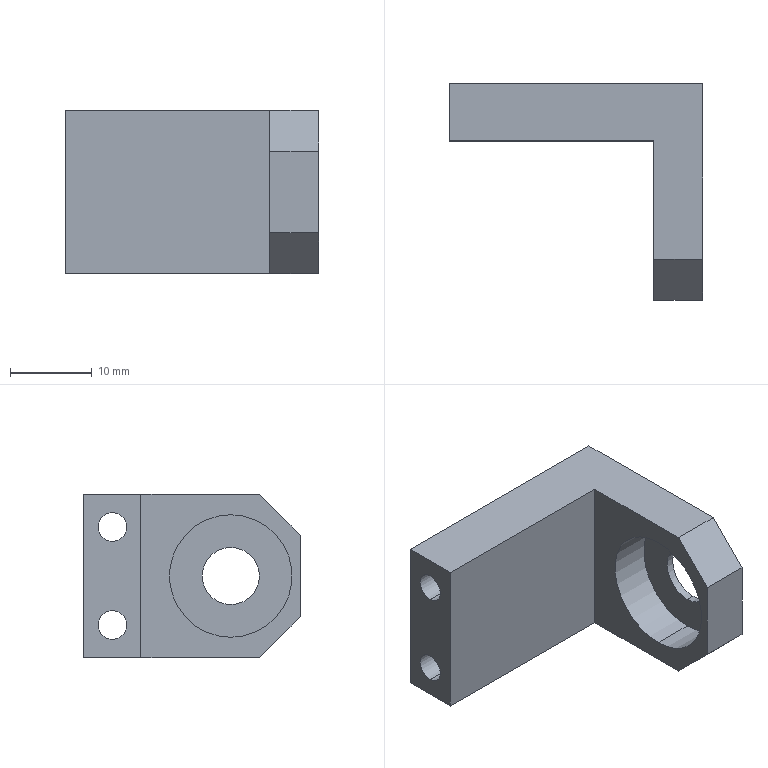Component | SolidWorks | AS-011-JG0130-1 | 1 solid | 19 faces | box 31 x 26.5 x 20 mm | volume 5011 mm3 | plane 11 | cylinder 8 | commonest cylinder face diameters 3.5 x4 15 x2 7 x2
build123d program:
from build123d import *

# Parameters (mm, degrees)
BOSS_EXTRUDE1_DEPTH = 20
SKETCH2_R           = 3.5
SKETCH2_R_2         = 1.75
CUT_EXTRUDE1_DEPTH  = 42
SKETCH5_R           = 7.5
CUT_EXTRUDE2_DEPTH  = 5
CHAMFER1_SIZE       = 5


with BuildPart() as part:
    # Sketch1 → Boss-Extrude1 (new body)
    with BuildSketch(Plane.XY):
        Polygon((-6, -7), (-6, -26.5), (0, -26.5), (0, 0), (-31, 0), (-31, -7), align=None)
    extrude(amount=-BOSS_EXTRUDE1_DEPTH)

    # Sketch2 → Cut-Extrude1 (cut)
    with BuildSketch(Plane(origin=(0, 0, 0), x_dir=(0, 0, -1), z_dir=(1, 0, 0))):
        with Locations((10, -18)):
            Circle(SKETCH2_R)
        with Locations((4, -3.5)):
            Circle(SKETCH2_R_2)
        with Locations((16, -3.5)):
            Circle(SKETCH2_R_2)
    extrude(amount=-CUT_EXTRUDE1_DEPTH, mode=Mode.SUBTRACT)

    # Sketch5 → Cut-Extrude2 (cut)
    with BuildSketch(Plane.ZY.offset(6)):
        with Locations((-10, -18)):
            Circle(SKETCH5_R)
    extrude(amount=-CUT_EXTRUDE2_DEPTH, mode=Mode.SUBTRACT)

    # Chamfer1
    chamfer1_edges = [part.edges().sort_by_distance(p)[0] for p in [
        (-3, -26.5, -20),
        (-3, -26.5, 0),
    ]]
    chamfer(chamfer1_edges, length=CHAMFER1_SIZE)


solid = part.part
STEP:
#1=COLOUR_RGB('',0.7922,0.8196,0.9333);
#2=FILL_AREA_STYLE_COLOUR('',#1);
#3=FILL_AREA_STYLE('',(#2));
#4=SURFACE_STYLE_FILL_AREA(#3);
#5=SURFACE_SIDE_STYLE('',(#4));
#6=SURFACE_STYLE_USAGE(.BOTH.,#5);
#7=PRESENTATION_STYLE_ASSIGNMENT((#6));
#8=CARTESIAN_POINT('',(-0.03937,-0.7087,-0.689));
#9=VERTEX_POINT('',#8);
#10=CARTESIAN_POINT('',(-0.03937,-0.7087,-0.09843));
#11=VERTEX_POINT('',#10);
#12=CARTESIAN_POINT('',(-0.03937,-0.7087,-0.3937));
#13=DIRECTION('',(-1.,0.,0.));
#14=DIRECTION('',(0.,0.,1.));
#15=AXIS2_PLACEMENT_3D('',#12,#13,#14);
#16=CIRCLE('',#15,0.2953);
#17=EDGE_CURVE('',#9,#11,#16,.T.);
#18=ORIENTED_EDGE('',*,*,#17,.F.);
#19=CARTESIAN_POINT('',(-0.2362,-0.7087,-0.689));
#20=VERTEX_POINT('',#19);
#21=CARTESIAN_POINT('',(-0.03937,-0.7087,-0.689));
#22=DIRECTION('',(-1.,0.,0.));
#23=VECTOR('',#22,39.37);
#24=LINE('',#21,#23);
#25=EDGE_CURVE('',#9,#20,#24,.T.);
#26=ORIENTED_EDGE('',*,*,#25,.T.);
#27=CARTESIAN_POINT('',(-0.2362,-0.7087,-0.09843));
#28=VERTEX_POINT('',#27);
#29=CARTESIAN_POINT('',(-0.2362,-0.7087,-0.3937));
#30=DIRECTION('',(-1.,0.,0.));
#31=DIRECTION('',(0.,0.,1.));
#32=AXIS2_PLACEMENT_3D('',#29,#30,#31);
#33=CIRCLE('',#32,0.2953);
#34=EDGE_CURVE('',#20,#28,#33,.T.);
#35=ORIENTED_EDGE('',*,*,#34,.T.);
#36=CARTESIAN_POINT('',(-0.03937,-0.7087,-0.09843));
#37=DIRECTION('',(-1.,0.,0.));
#38=VECTOR('',#37,39.37);
#39=LINE('',#36,#38);
#40=EDGE_CURVE('',#11,#28,#39,.T.);
#41=ORIENTED_EDGE('',*,*,#40,.F.);
#42=EDGE_LOOP('',(#18,#26,#35,#41));
#43=FACE_OUTER_BOUND('',#42,.T.);
#44=CARTESIAN_POINT('',(-0.03937,-0.7087,-0.3937));
#45=DIRECTION('',(-1.,0.,0.));
#46=DIRECTION('',(0.,0.,1.));
#47=AXIS2_PLACEMENT_3D('',#44,#45,#46);
#48=CYLINDRICAL_SURFACE('',#47,0.2953);
#49=ADVANCED_FACE('',(#43),#48,.F.);
#50=CARTESIAN_POINT('',(-1.22,-0.1378,-0.6988));
#51=VERTEX_POINT('',#50);
#52=CARTESIAN_POINT('',(-1.22,-0.1378,-0.561));
#53=VERTEX_POINT('',#52);
#54=CARTESIAN_POINT('',(-1.22,-0.1378,-0.6299));
#55=DIRECTION('',(-1.,0.,0.));
#56=DIRECTION('',(0.,0.,1.));
#57=AXIS2_PLACEMENT_3D('',#54,#55,#56);
#58=CIRCLE('',#57,0.0689);
#59=EDGE_CURVE('',#51,#53,#58,.T.);
#60=ORIENTED_EDGE('',*,*,#59,.T.);
#61=CARTESIAN_POINT('',(0.,-0.1378,-0.561));
#62=VERTEX_POINT('',#61);
#63=CARTESIAN_POINT('',(-1.654,-0.1378,-0.561));
#64=DIRECTION('',(1.,0.,0.));
#65=VECTOR('',#64,39.37);
#66=LINE('',#63,#65);
#67=EDGE_CURVE('',#53,#62,#66,.T.);
#68=ORIENTED_EDGE('',*,*,#67,.T.);
#69=CARTESIAN_POINT('',(0.,-0.1378,-0.6988));
#70=VERTEX_POINT('',#69);
#71=CARTESIAN_POINT('',(0.,-0.1378,-0.6299));
#72=DIRECTION('',(1.,0.,0.));
#73=DIRECTION('',(0.,0.,-1.));
#74=AXIS2_PLACEMENT_3D('',#71,#72,#73);
#75=CIRCLE('',#74,0.0689);
#76=EDGE_CURVE('',#62,#70,#75,.T.);
#77=ORIENTED_EDGE('',*,*,#76,.T.);
#78=CARTESIAN_POINT('',(-1.654,-0.1378,-0.6988));
#79=DIRECTION('',(1.,0.,0.));
#80=VECTOR('',#79,39.37);
#81=LINE('',#78,#80);
#82=EDGE_CURVE('',#51,#70,#81,.T.);
#83=ORIENTED_EDGE('',*,*,#82,.F.);
#84=EDGE_LOOP('',(#60,#68,#77,#83));
#85=FACE_OUTER_BOUND('',#84,.T.);
#86=CARTESIAN_POINT('',(-1.654,-0.1378,-0.6299));
#87=DIRECTION('',(1.,0.,0.));
#88=DIRECTION('',(0.,0.,-1.));
#89=AXIS2_PLACEMENT_3D('',#86,#87,#88);
#90=CYLINDRICAL_SURFACE('',#89,0.0689);
#91=ADVANCED_FACE('',(#85),#90,.F.);
#92=CARTESIAN_POINT('',(-1.22,-0.1378,-0.2264));
#93=VERTEX_POINT('',#92);
#94=CARTESIAN_POINT('',(-1.22,-0.1378,-0.08858));
#95=VERTEX_POINT('',#94);
#96=CARTESIAN_POINT('',(-1.22,-0.1378,-0.1575));
#97=DIRECTION('',(-1.,0.,0.));
#98=DIRECTION('',(0.,0.,1.));
#99=AXIS2_PLACEMENT_3D('',#96,#97,#98);
#100=CIRCLE('',#99,0.0689);
#101=EDGE_CURVE('',#93,#95,#100,.T.);
#102=ORIENTED_EDGE('',*,*,#101,.T.);
#103=CARTESIAN_POINT('',(0.,-0.1378,-0.08858));
#104=VERTEX_POINT('',#103);
#105=CARTESIAN_POINT('',(-1.654,-0.1378,-0.08858));
#106=DIRECTION('',(1.,0.,0.));
#107=VECTOR('',#106,39.37);
#108=LINE('',#105,#107);
#109=EDGE_CURVE('',#95,#104,#108,.T.);
#110=ORIENTED_EDGE('',*,*,#109,.T.);
#111=CARTESIAN_POINT('',(0.,-0.1378,-0.2264));
#112=VERTEX_POINT('',#111);
#113=CARTESIAN_POINT('',(0.,-0.1378,-0.1575));
#114=DIRECTION('',(1.,0.,0.));
#115=DIRECTION('',(0.,0.,-1.));
#116=AXIS2_PLACEMENT_3D('',#113,#114,#115);
#117=CIRCLE('',#116,0.0689);
#118=EDGE_CURVE('',#104,#112,#117,.T.);
#119=ORIENTED_EDGE('',*,*,#118,.T.);
#120=CARTESIAN_POINT('',(-1.654,-0.1378,-0.2264));
#121=DIRECTION('',(1.,0.,0.));
#122=VECTOR('',#121,39.37);
#123=LINE('',#120,#122);
#124=EDGE_CURVE('',#93,#112,#123,.T.);
#125=ORIENTED_EDGE('',*,*,#124,.F.);
#126=EDGE_LOOP('',(#102,#110,#119,#125));
#127=FACE_OUTER_BOUND('',#126,.T.);
#128=CARTESIAN_POINT('',(-1.654,-0.1378,-0.1575));
#129=DIRECTION('',(1.,0.,0.));
#130=DIRECTION('',(0.,0.,-1.));
#131=AXIS2_PLACEMENT_3D('',#128,#129,#130);
#132=CYLINDRICAL_SURFACE('',#131,0.0689);
#133=ADVANCED_FACE('',(#127),#132,.F.);
#134=CARTESIAN_POINT('',(-0.03937,-0.7087,-0.2559));
#135=VERTEX_POINT('',#134);
#136=CARTESIAN_POINT('',(-0.03937,-0.7087,-0.5315));
#137=VERTEX_POINT('',#136);
#138=CARTESIAN_POINT('',(-0.03937,-0.7087,-0.3937));
#139=DIRECTION('',(1.,0.,0.));
#140=DIRECTION('',(0.,0.,1.));
#141=AXIS2_PLACEMENT_3D('',#138,#139,#140);
#142=CIRCLE('',#141,0.1378);
#143=EDGE_CURVE('',#135,#137,#142,.T.);
#144=ORIENTED_EDGE('',*,*,#143,.F.);
#145=CARTESIAN_POINT('',(0.,-0.7087,-0.2559));
#146=VERTEX_POINT('',#145);
#147=CARTESIAN_POINT('',(-1.654,-0.7087,-0.2559));
#148=DIRECTION('',(1.,0.,0.));
#149=VECTOR('',#148,39.37);
#150=LINE('',#147,#149);
#151=EDGE_CURVE('',#135,#146,#150,.T.);
#152=ORIENTED_EDGE('',*,*,#151,.T.);
#153=CARTESIAN_POINT('',(0.,-0.7087,-0.5315));
#154=VERTEX_POINT('',#153);
#155=CARTESIAN_POINT('',(0.,-0.7087,-0.3937));
#156=DIRECTION('',(1.,0.,0.));
#157=DIRECTION('',(0.,0.,-1.));
#158=AXIS2_PLACEMENT_3D('',#155,#156,#157);
#159=CIRCLE('',#158,0.1378);
#160=EDGE_CURVE('',#146,#154,#159,.T.);
#161=ORIENTED_EDGE('',*,*,#160,.T.);
#162=CARTESIAN_POINT('',(-1.654,-0.7087,-0.5315));
#163=DIRECTION('',(1.,0.,0.));
#164=VECTOR('',#163,39.37);
#165=LINE('',#162,#164);
#166=EDGE_CURVE('',#137,#154,#165,.T.);
#167=ORIENTED_EDGE('',*,*,#166,.F.);
#168=EDGE_LOOP('',(#144,#152,#161,#167));
#169=FACE_OUTER_BOUND('',#168,.T.);
#170=CARTESIAN_POINT('',(-1.654,-0.7087,-0.3937));
#171=DIRECTION('',(1.,0.,0.));
#172=DIRECTION('',(0.,0.,-1.));
#173=AXIS2_PLACEMENT_3D('',#170,#171,#172);
#174=CYLINDRICAL_SURFACE('',#173,0.1378);
#175=ADVANCED_FACE('',(#169),#174,.F.);
#176=ORIENTED_EDGE('',*,*,#151,.F.);
#177=CARTESIAN_POINT('',(-0.03937,-0.7087,-0.3937));
#178=DIRECTION('',(1.,0.,0.));
#179=DIRECTION('',(0.,0.,1.));
#180=AXIS2_PLACEMENT_3D('',#177,#178,#179);
#181=CIRCLE('',#180,0.1378);
#182=EDGE_CURVE('',#137,#135,#181,.T.);
#183=ORIENTED_EDGE('',*,*,#182,.F.);
#184=ORIENTED_EDGE('',*,*,#166,.T.);
#185=CARTESIAN_POINT('',(0.,-0.7087,-0.3937));
#186=DIRECTION('',(1.,0.,0.));
#187=DIRECTION('',(0.,0.,-1.));
#188=AXIS2_PLACEMENT_3D('',#185,#186,#187);
#189=CIRCLE('',#188,0.1378);
#190=EDGE_CURVE('',#154,#146,#189,.T.);
#191=ORIENTED_EDGE('',*,*,#190,.T.);
#192=EDGE_LOOP('',(#176,#183,#184,#191));
#193=FACE_OUTER_BOUND('',#192,.T.);
#194=CARTESIAN_POINT('',(-1.654,-0.7087,-0.3937));
#195=DIRECTION('',(1.,0.,0.));
#196=DIRECTION('',(0.,0.,-1.));
#197=AXIS2_PLACEMENT_3D('',#194,#195,#196);
#198=CYLINDRICAL_SURFACE('',#197,0.1378);
#199=ADVANCED_FACE('',(#193),#198,.F.);
#200=CARTESIAN_POINT('',(-1.22,-0.2756,0.));
#201=VERTEX_POINT('',#200);
#202=CARTESIAN_POINT('',(-0.2362,-0.2756,0.));
#203=VERTEX_POINT('',#202);
#204=CARTESIAN_POINT('',(-1.22,-0.2756,0.));
#205=DIRECTION('',(1.,0.,0.));
#206=VECTOR('',#205,39.37);
#207=LINE('',#204,#206);
#208=EDGE_CURVE('',#201,#203,#207,.T.);
#209=ORIENTED_EDGE('',*,*,#208,.F.);
#210=CARTESIAN_POINT('',(-1.22,-0.2756,-0.7874));
#211=VERTEX_POINT('',#210);
#212=CARTESIAN_POINT('',(-1.22,-0.2756,-0.7874));
#213=DIRECTION('',(0.,0.,1.));
#214=VECTOR('',#213,39.37);
#215=LINE('',#212,#214);
#216=EDGE_CURVE('',#211,#201,#215,.T.);
#217=ORIENTED_EDGE('',*,*,#216,.F.);
#218=CARTESIAN_POINT('',(-0.2362,-0.2756,-0.7874));
#219=VERTEX_POINT('',#218);
#220=CARTESIAN_POINT('',(-1.22,-0.2756,-0.7874));
#221=DIRECTION('',(1.,0.,0.));
#222=VECTOR('',#221,39.37);
#223=LINE('',#220,#222);
#224=EDGE_CURVE('',#211,#219,#223,.T.);
#225=ORIENTED_EDGE('',*,*,#224,.T.);
#226=CARTESIAN_POINT('',(-0.2362,-0.2756,-0.7874));
#227=DIRECTION('',(0.,0.,1.));
#228=VECTOR('',#227,39.37);
#229=LINE('',#226,#228);
#230=EDGE_CURVE('',#219,#203,#229,.T.);
#231=ORIENTED_EDGE('',*,*,#230,.T.);
#232=EDGE_LOOP('',(#209,#217,#225,#231));
#233=FACE_OUTER_BOUND('',#232,.T.);
#234=CARTESIAN_POINT('',(-1.22,-0.2756,-0.7874));
#235=DIRECTION('',(0.,-1.,0.));
#236=DIRECTION('',(0.,0.,-1.));
#237=AXIS2_PLACEMENT_3D('',#234,#235,#236);
#238=PLANE('',#237);
#239=ADVANCED_FACE('',(#233),#238,.T.);
#240=ORIENTED_EDGE('',*,*,#59,.F.);
#241=CARTESIAN_POINT('',(-1.22,-0.1378,-0.6299));
#242=DIRECTION('',(-1.,0.,0.));
#243=DIRECTION('',(0.,0.,1.));
#244=AXIS2_PLACEMENT_3D('',#241,#242,#243);
#245=CIRCLE('',#244,0.0689);
#246=EDGE_CURVE('',#53,#51,#245,.T.);
#247=ORIENTED_EDGE('',*,*,#246,.F.);
#248=EDGE_LOOP('',(#240,#247));
#249=FACE_BOUND('',#248,.T.);
#250=ORIENTED_EDGE('',*,*,#101,.F.);
#251=CARTESIAN_POINT('',(-1.22,-0.1378,-0.1575));
#252=DIRECTION('',(-1.,0.,0.));
#253=DIRECTION('',(0.,0.,1.));
#254=AXIS2_PLACEMENT_3D('',#251,#252,#253);
#255=CIRCLE('',#254,0.0689);
#256=EDGE_CURVE('',#95,#93,#255,.T.);
#257=ORIENTED_EDGE('',*,*,#256,.F.);
#258=EDGE_LOOP('',(#250,#257));
#259=FACE_BOUND('',#258,.T.);
#260=CARTESIAN_POINT('',(-1.22,0.,0.));
#261=VERTEX_POINT('',#260);
#262=CARTESIAN_POINT('',(-1.22,-0.2756,0.));
#263=DIRECTION('',(0.,-1.,0.));
#264=VECTOR('',#263,39.37);
#265=LINE('',#262,#264);
#266=EDGE_CURVE('',#261,#201,#265,.T.);
#267=ORIENTED_EDGE('',*,*,#266,.F.);
#268=CARTESIAN_POINT('',(-1.22,0.,-0.7874));
#269=VERTEX_POINT('',#268);
#270=CARTESIAN_POINT('',(-1.22,0.,-0.7874));
#271=DIRECTION('',(0.,0.,1.));
#272=VECTOR('',#271,39.37);
#273=LINE('',#270,#272);
#274=EDGE_CURVE('',#269,#261,#273,.T.);
#275=ORIENTED_EDGE('',*,*,#274,.F.);
#276=CARTESIAN_POINT('',(-1.22,-0.2756,-0.7874));
#277=DIRECTION('',(0.,-1.,0.));
#278=VECTOR('',#277,39.37);
#279=LINE('',#276,#278);
#280=EDGE_CURVE('',#269,#211,#279,.T.);
#281=ORIENTED_EDGE('',*,*,#280,.T.);
#282=ORIENTED_EDGE('',*,*,#216,.T.);
#283=EDGE_LOOP('',(#267,#275,#281,#282));
#284=FACE_OUTER_BOUND('',#283,.T.);
#285=CARTESIAN_POINT('',(-1.22,-0.2756,-0.7874));
#286=DIRECTION('',(-1.,0.,0.));
#287=DIRECTION('',(0.,0.,1.));
#288=AXIS2_PLACEMENT_3D('',#285,#286,#287);
#289=PLANE('',#288);
#290=ADVANCED_FACE('',(#249,#259,#284),#289,.T.);
#291=CARTESIAN_POINT('',(0.,0.,0.));
#292=VERTEX_POINT('',#291);
#293=CARTESIAN_POINT('',(0.,0.,0.));
#294=DIRECTION('',(-1.,0.,0.));
#295=VECTOR('',#294,39.37);
#296=LINE('',#293,#295);
#297=EDGE_CURVE('',#292,#261,#296,.T.);
#298=ORIENTED_EDGE('',*,*,#297,.F.);
#299=CARTESIAN_POINT('',(0.,0.,-0.7874));
#300=VERTEX_POINT('',#299);
#301=CARTESIAN_POINT('',(0.,0.,-0.7874));
#302=DIRECTION('',(0.,0.,1.));
#303=VECTOR('',#302,39.37);
#304=LINE('',#301,#303);
#305=EDGE_CURVE('',#300,#292,#304,.T.);
#306=ORIENTED_EDGE('',*,*,#305,.F.);
#307=CARTESIAN_POINT('',(0.,0.,-0.7874));
#308=DIRECTION('',(-1.,0.,0.));
#309=VECTOR('',#308,39.37);
#310=LINE('',#307,#309);
#311=EDGE_CURVE('',#300,#269,#310,.T.);
#312=ORIENTED_EDGE('',*,*,#311,.T.);
#313=ORIENTED_EDGE('',*,*,#274,.T.);
#314=EDGE_LOOP('',(#298,#306,#312,#313));
#315=FACE_OUTER_BOUND('',#314,.T.);
#316=CARTESIAN_POINT('',(0.,0.,-0.7874));
#317=DIRECTION('',(0.,1.,0.));
#318=DIRECTION('',(0.,0.,1.));
#319=AXIS2_PLACEMENT_3D('',#316,#317,#318);
#320=PLANE('',#319);
#321=ADVANCED_FACE('',(#315),#320,.T.);
#322=CARTESIAN_POINT('',(0.,-0.1378,-0.6299));
#323=DIRECTION('',(1.,0.,0.));
#324=DIRECTION('',(0.,0.,-1.));
#325=AXIS2_PLACEMENT_3D('',#322,#323,#324);
#326=CIRCLE('',#325,0.0689);
#327=EDGE_CURVE('',#70,#62,#326,.T.);
#328=ORIENTED_EDGE('',*,*,#327,.F.);
#329=ORIENTED_EDGE('',*,*,#76,.F.);
#330=EDGE_LOOP('',(#328,#329));
#331=FACE_BOUND('',#330,.T.);
#332=CARTESIAN_POINT('',(0.,-0.1378,-0.1575));
#333=DIRECTION('',(1.,0.,0.));
#334=DIRECTION('',(0.,0.,-1.));
#335=AXIS2_PLACEMENT_3D('',#332,#333,#334);
#336=CIRCLE('',#335,0.0689);
#337=EDGE_CURVE('',#112,#104,#336,.T.);
#338=ORIENTED_EDGE('',*,*,#337,.F.);
#339=ORIENTED_EDGE('',*,*,#118,.F.);
#340=EDGE_LOOP('',(#338,#339));
#341=FACE_BOUND('',#340,.T.);
#342=ORIENTED_EDGE('',*,*,#190,.F.);
#343=ORIENTED_EDGE('',*,*,#160,.F.);
#344=EDGE_LOOP('',(#342,#343));
#345=FACE_BOUND('',#344,.T.);
#346=CARTESIAN_POINT('',(0.,-1.043,-0.5906));
#347=VERTEX_POINT('',#346);
#348=CARTESIAN_POINT('',(0.,-1.043,-0.1969));
#349=VERTEX_POINT('',#348);
#350=CARTESIAN_POINT('',(0.,-1.043,-0.7874));
#351=DIRECTION('',(0.,0.,1.));
#352=VECTOR('',#351,39.37);
#353=LINE('',#350,#352);
#354=EDGE_CURVE('',#347,#349,#353,.T.);
#355=ORIENTED_EDGE('',*,*,#354,.F.);
#356=CARTESIAN_POINT('',(0.,-0.8465,-0.7874));
#357=VERTEX_POINT('',#356);
#358=CARTESIAN_POINT('',(0.,-0.4232,-1.211));
#359=DIRECTION('',(0.,0.7071,-0.7071));
#360=VECTOR('',#359,39.37);
#361=LINE('',#358,#360);
#362=EDGE_CURVE('',#347,#357,#361,.T.);
#363=ORIENTED_EDGE('',*,*,#362,.T.);
#364=CARTESIAN_POINT('',(0.,0.,-0.7874));
#365=DIRECTION('',(0.,1.,0.));
#366=VECTOR('',#365,39.37);
#367=LINE('',#364,#366);
#368=EDGE_CURVE('',#357,#300,#367,.T.);
#369=ORIENTED_EDGE('',*,*,#368,.T.);
#370=ORIENTED_EDGE('',*,*,#305,.T.);
#371=CARTESIAN_POINT('',(0.,-0.8465,-0.));
#372=VERTEX_POINT('',#371);
#373=CARTESIAN_POINT('',(0.,0.,0.));
#374=DIRECTION('',(0.,1.,0.));
#375=VECTOR('',#374,39.37);
#376=LINE('',#373,#375);
#377=EDGE_CURVE('',#372,#292,#376,.T.);
#378=ORIENTED_EDGE('',*,*,#377,.F.);
#379=CARTESIAN_POINT('',(0.,-0.8169,0.02953));
#380=DIRECTION('',(0.,-0.7071,-0.7071));
#381=VECTOR('',#380,39.37);
#382=LINE('',#379,#381);
#383=EDGE_CURVE('',#372,#349,#382,.T.);
#384=ORIENTED_EDGE('',*,*,#383,.T.);
#385=EDGE_LOOP('',(#355,#363,#369,#370,#378,#384));
#386=FACE_OUTER_BOUND('',#385,.T.);
#387=CARTESIAN_POINT('',(0.,0.,-0.7874));
#388=DIRECTION('',(1.,0.,0.));
#389=DIRECTION('',(0.,0.,-1.));
#390=AXIS2_PLACEMENT_3D('',#387,#388,#389);
#391=PLANE('',#390);
#392=ADVANCED_FACE('',(#331,#341,#345,#386),#391,.T.);
#393=CARTESIAN_POINT('',(-0.2362,-1.043,-0.5906));
#394=VERTEX_POINT('',#393);
#395=CARTESIAN_POINT('',(-0.2362,-1.043,-0.1969));
#396=VERTEX_POINT('',#395);
#397=CARTESIAN_POINT('',(-0.2362,-1.043,-0.7874));
#398=DIRECTION('',(0.,0.,1.));
#399=VECTOR('',#398,39.37);
#400=LINE('',#397,#399);
#401=EDGE_CURVE('',#394,#396,#400,.T.);
#402=ORIENTED_EDGE('',*,*,#401,.F.);
#403=CARTESIAN_POINT('',(0.,-1.043,-0.5906));
#404=DIRECTION('',(1.,0.,0.));
#405=VECTOR('',#404,39.37);
#406=LINE('',#403,#405);
#407=EDGE_CURVE('',#394,#347,#406,.T.);
#408=ORIENTED_EDGE('',*,*,#407,.T.);
#409=ORIENTED_EDGE('',*,*,#354,.T.);
#410=CARTESIAN_POINT('',(-0.2362,-1.043,-0.1969));
#411=DIRECTION('',(-1.,0.,0.));
#412=VECTOR('',#411,39.37);
#413=LINE('',#410,#412);
#414=EDGE_CURVE('',#349,#396,#413,.T.);
#415=ORIENTED_EDGE('',*,*,#414,.T.);
#416=EDGE_LOOP('',(#402,#408,#409,#415));
#417=FACE_OUTER_BOUND('',#416,.T.);
#418=CARTESIAN_POINT('',(0.,-1.043,-0.7874));
#419=DIRECTION('',(0.,-1.,0.));
#420=DIRECTION('',(0.,0.,-1.));
#421=AXIS2_PLACEMENT_3D('',#418,#419,#420);
#422=PLANE('',#421);
#423=ADVANCED_FACE('',(#417),#422,.T.);
#424=CARTESIAN_POINT('',(-0.2362,-0.7087,-0.3937));
#425=DIRECTION('',(-1.,0.,0.));
#426=DIRECTION('',(0.,0.,1.));
#427=AXIS2_PLACEMENT_3D('',#424,#425,#426);
#428=CIRCLE('',#427,0.2953);
#429=EDGE_CURVE('',#28,#20,#428,.T.);
#430=ORIENTED_EDGE('',*,*,#429,.F.);
#431=ORIENTED_EDGE('',*,*,#34,.F.);
#432=EDGE_LOOP('',(#430,#431));
#433=FACE_BOUND('',#432,.T.);
#434=CARTESIAN_POINT('',(-0.2362,-0.8465,-0.7874));
#435=VERTEX_POINT('',#434);
#436=CARTESIAN_POINT('',(-0.2362,-0.2756,-0.7874));
#437=DIRECTION('',(0.,-1.,0.));
#438=VECTOR('',#437,39.37);
#439=LINE('',#436,#438);
#440=EDGE_CURVE('',#219,#435,#439,.T.);
#441=ORIENTED_EDGE('',*,*,#440,.T.);
#442=CARTESIAN_POINT('',(-0.2362,-0.561,-1.073));
#443=DIRECTION('',(0.,-0.7071,0.7071));
#444=VECTOR('',#443,39.37);
#445=LINE('',#442,#444);
#446=EDGE_CURVE('',#435,#394,#445,.T.);
#447=ORIENTED_EDGE('',*,*,#446,.T.);
#448=ORIENTED_EDGE('',*,*,#401,.T.);
#449=CARTESIAN_POINT('',(-0.2362,-0.8465,-0.));
#450=VERTEX_POINT('',#449);
#451=CARTESIAN_POINT('',(-0.2362,-0.9547,-0.1083));
#452=DIRECTION('',(0.,0.7071,0.7071));
#453=VECTOR('',#452,39.37);
#454=LINE('',#451,#453);
#455=EDGE_CURVE('',#396,#450,#454,.T.);
#456=ORIENTED_EDGE('',*,*,#455,.T.);
#457=CARTESIAN_POINT('',(-0.2362,-0.2756,0.));
#458=DIRECTION('',(0.,-1.,0.));
#459=VECTOR('',#458,39.37);
#460=LINE('',#457,#459);
#461=EDGE_CURVE('',#203,#450,#460,.T.);
#462=ORIENTED_EDGE('',*,*,#461,.F.);
#463=ORIENTED_EDGE('',*,*,#230,.F.);
#464=EDGE_LOOP('',(#441,#447,#448,#456,#462,#463));
#465=FACE_OUTER_BOUND('',#464,.T.);
#466=CARTESIAN_POINT('',(-0.2362,-0.2756,-0.7874));
#467=DIRECTION('',(-1.,0.,0.));
#468=DIRECTION('',(0.,0.,1.));
#469=AXIS2_PLACEMENT_3D('',#466,#467,#468);
#470=PLANE('',#469);
#471=ADVANCED_FACE('',(#433,#465),#470,.T.);
#472=ORIENTED_EDGE('',*,*,#368,.F.);
#473=CARTESIAN_POINT('',(0.,-0.8465,-0.7874));
#474=DIRECTION('',(-1.,0.,0.));
#475=VECTOR('',#474,39.37);
#476=LINE('',#473,#475);
#477=EDGE_CURVE('',#357,#435,#476,.T.);
#478=ORIENTED_EDGE('',*,*,#477,.T.);
#479=ORIENTED_EDGE('',*,*,#440,.F.);
#480=ORIENTED_EDGE('',*,*,#224,.F.);
#481=ORIENTED_EDGE('',*,*,#280,.F.);
#482=ORIENTED_EDGE('',*,*,#311,.F.);
#483=EDGE_LOOP('',(#472,#478,#479,#480,#481,#482));
#484=FACE_OUTER_BOUND('',#483,.T.);
#485=CARTESIAN_POINT('',(0.,0.,-0.7874));
#486=DIRECTION('',(0.,0.,-1.));
#487=DIRECTION('',(-1.,0.,0.));
#488=AXIS2_PLACEMENT_3D('',#485,#486,#487);
#489=PLANE('',#488);
#490=ADVANCED_FACE('',(#484),#489,.T.);
#491=ORIENTED_EDGE('',*,*,#461,.T.);
#492=CARTESIAN_POINT('',(0.,-0.8465,0.));
#493=DIRECTION('',(1.,0.,0.));
#494=VECTOR('',#493,39.37);
#495=LINE('',#492,#494);
#496=EDGE_CURVE('',#450,#372,#495,.T.);
#497=ORIENTED_EDGE('',*,*,#496,.T.);
#498=ORIENTED_EDGE('',*,*,#377,.T.);
#499=ORIENTED_EDGE('',*,*,#297,.T.);
#500=ORIENTED_EDGE('',*,*,#266,.T.);
#501=ORIENTED_EDGE('',*,*,#208,.T.);
#502=EDGE_LOOP('',(#491,#497,#498,#499,#500,#501));
#503=FACE_OUTER_BOUND('',#502,.T.);
#504=CARTESIAN_POINT('',(0.,0.,0.));
#505=DIRECTION('',(0.,0.,-1.));
#506=DIRECTION('',(-1.,0.,0.));
#507=AXIS2_PLACEMENT_3D('',#504,#505,#506);
#508=PLANE('',#507);
#509=ADVANCED_FACE('',(#503),#508,.F.);
#510=ORIENTED_EDGE('',*,*,#109,.F.);
#511=ORIENTED_EDGE('',*,*,#256,.T.);
#512=ORIENTED_EDGE('',*,*,#124,.T.);
#513=ORIENTED_EDGE('',*,*,#337,.T.);
#514=EDGE_LOOP('',(#510,#511,#512,#513));
#515=FACE_OUTER_BOUND('',#514,.T.);
#516=CARTESIAN_POINT('',(-1.654,-0.1378,-0.1575));
#517=DIRECTION('',(1.,0.,0.));
#518=DIRECTION('',(0.,0.,-1.));
#519=AXIS2_PLACEMENT_3D('',#516,#517,#518);
#520=CYLINDRICAL_SURFACE('',#519,0.0689);
#521=ADVANCED_FACE('',(#515),#520,.F.);
#522=ORIENTED_EDGE('',*,*,#67,.F.);
#523=ORIENTED_EDGE('',*,*,#246,.T.);
#524=ORIENTED_EDGE('',*,*,#82,.T.);
#525=ORIENTED_EDGE('',*,*,#327,.T.);
#526=EDGE_LOOP('',(#522,#523,#524,#525));
#527=FACE_OUTER_BOUND('',#526,.T.);
#528=CARTESIAN_POINT('',(-1.654,-0.1378,-0.6299));
#529=DIRECTION('',(1.,0.,0.));
#530=DIRECTION('',(0.,0.,-1.));
#531=AXIS2_PLACEMENT_3D('',#528,#529,#530);
#532=CYLINDRICAL_SURFACE('',#531,0.0689);
#533=ADVANCED_FACE('',(#527),#532,.F.);
#534=CARTESIAN_POINT('',(-0.03937,-0.7087,-0.3937));
#535=DIRECTION('',(-1.,0.,0.));
#536=DIRECTION('',(0.,0.,1.));
#537=AXIS2_PLACEMENT_3D('',#534,#535,#536);
#538=CIRCLE('',#537,0.2953);
#539=EDGE_CURVE('',#11,#9,#538,.T.);
#540=ORIENTED_EDGE('',*,*,#539,.T.);
#541=ORIENTED_EDGE('',*,*,#17,.T.);
#542=EDGE_LOOP('',(#540,#541));
#543=FACE_OUTER_BOUND('',#542,.T.);
#544=ORIENTED_EDGE('',*,*,#182,.T.);
#545=ORIENTED_EDGE('',*,*,#143,.T.);
#546=EDGE_LOOP('',(#544,#545));
#547=FACE_BOUND('',#546,.T.);
#548=CARTESIAN_POINT('',(-0.03937,-0.7087,-0.3937));
#549=DIRECTION('',(-1.,0.,0.));
#550=DIRECTION('',(0.,0.,1.));
#551=AXIS2_PLACEMENT_3D('',#548,#549,#550);
#552=PLANE('',#551);
#553=ADVANCED_FACE('',(#543,#547),#552,.T.);
#554=ORIENTED_EDGE('',*,*,#25,.F.);
#555=ORIENTED_EDGE('',*,*,#539,.F.);
#556=ORIENTED_EDGE('',*,*,#40,.T.);
#557=ORIENTED_EDGE('',*,*,#429,.T.);
#558=EDGE_LOOP('',(#554,#555,#556,#557));
#559=FACE_OUTER_BOUND('',#558,.T.);
#560=CARTESIAN_POINT('',(-0.03937,-0.7087,-0.3937));
#561=DIRECTION('',(-1.,0.,0.));
#562=DIRECTION('',(0.,0.,1.));
#563=AXIS2_PLACEMENT_3D('',#560,#561,#562);
#564=CYLINDRICAL_SURFACE('',#563,0.2953);
#565=ADVANCED_FACE('',(#559),#564,.F.);
#566=ORIENTED_EDGE('',*,*,#446,.F.);
#567=ORIENTED_EDGE('',*,*,#477,.F.);
#568=ORIENTED_EDGE('',*,*,#362,.F.);
#569=ORIENTED_EDGE('',*,*,#407,.F.);
#570=EDGE_LOOP('',(#566,#567,#568,#569));
#571=FACE_OUTER_BOUND('',#570,.T.);
#572=CARTESIAN_POINT('',(0.,-1.043,-0.5906));
#573=DIRECTION('',(0.,0.7071,0.7071));
#574=DIRECTION('',(1.,0.,0.));
#575=AXIS2_PLACEMENT_3D('',#572,#573,#574);
#576=PLANE('',#575);
#577=ADVANCED_FACE('',(#571),#576,.F.);
#578=ORIENTED_EDGE('',*,*,#455,.F.);
#579=ORIENTED_EDGE('',*,*,#414,.F.);
#580=ORIENTED_EDGE('',*,*,#383,.F.);
#581=ORIENTED_EDGE('',*,*,#496,.F.);
#582=EDGE_LOOP('',(#578,#579,#580,#581));
#583=FACE_OUTER_BOUND('',#582,.T.);
#584=CARTESIAN_POINT('',(0.,-0.8465,0.));
#585=DIRECTION('',(0.,-0.7071,0.7071));
#586=DIRECTION('',(-1.,0.,0.));
#587=AXIS2_PLACEMENT_3D('',#584,#585,#586);
#588=PLANE('',#587);
#589=ADVANCED_FACE('',(#583),#588,.T.);
#590=CLOSED_SHELL('',(#49,#91,#133,#175,#199,#239,#290,#321,#392,#423,#471,#490,#509,#521,#533,#553,#565,#577,#589));
#591=MANIFOLD_SOLID_BREP('',#590);
#592=STYLED_ITEM('',(#7),#591);
#593=PRESENTATION_LAYER_ASSIGNMENT('','',(#592));
#594=(LENGTH_UNIT()NAMED_UNIT(*)SI_UNIT($,.METRE.));
#595=LENGTH_MEASURE_WITH_UNIT(LENGTH_MEASURE(0.0254),#594);
#596=DIMENSIONAL_EXPONENTS(1.,0.,0.,0.,0.,0.,0.);
#597=(CONVERSION_BASED_UNIT('',#595)LENGTH_UNIT()NAMED_UNIT(#596));
#598=UNCERTAINTY_MEASURE_WITH_UNIT(LENGTH_MEASURE(0.00001),#597,'','');
#599=(NAMED_UNIT(*)PLANE_ANGLE_UNIT()SI_UNIT($,.RADIAN.));
#600=(NAMED_UNIT(*)SI_UNIT($,.STERADIAN.)SOLID_ANGLE_UNIT());
#601=(GEOMETRIC_REPRESENTATION_CONTEXT(3)GLOBAL_UNCERTAINTY_ASSIGNED_CONTEXT((#598))GLOBAL_UNIT_ASSIGNED_CONTEXT((#597,#599,#600))REPRESENTATION_CONTEXT('',''));
#602=MECHANICAL_DESIGN_GEOMETRIC_PRESENTATION_REPRESENTATION('',(#592),#601);
#603=CARTESIAN_POINT('',(0.,0.,0.));
#604=DIRECTION('',(0.,0.,1.));
#605=DIRECTION('',(1.,0.,0.));
#606=AXIS2_PLACEMENT_3D('',#603,#604,#605);
#607=(LENGTH_UNIT()NAMED_UNIT(*)SI_UNIT($,.METRE.));
#608=LENGTH_MEASURE_WITH_UNIT(LENGTH_MEASURE(0.0254),#607);
#609=DIMENSIONAL_EXPONENTS(1.,0.,0.,0.,0.,0.,0.);
#610=(CONVERSION_BASED_UNIT('',#608)LENGTH_UNIT()NAMED_UNIT(#609));
#611=UNCERTAINTY_MEASURE_WITH_UNIT(LENGTH_MEASURE(0.00001),#610,'','');
#612=(NAMED_UNIT(*)PLANE_ANGLE_UNIT()SI_UNIT($,.RADIAN.));
#613=(NAMED_UNIT(*)SI_UNIT($,.STERADIAN.)SOLID_ANGLE_UNIT());
#614=(GEOMETRIC_REPRESENTATION_CONTEXT(3)GLOBAL_UNCERTAINTY_ASSIGNED_CONTEXT((#611))GLOBAL_UNIT_ASSIGNED_CONTEXT((#610,#612,#613))REPRESENTATION_CONTEXT('',''));
#615=ADVANCED_BREP_SHAPE_REPRESENTATION('',(#591,#606),#614);